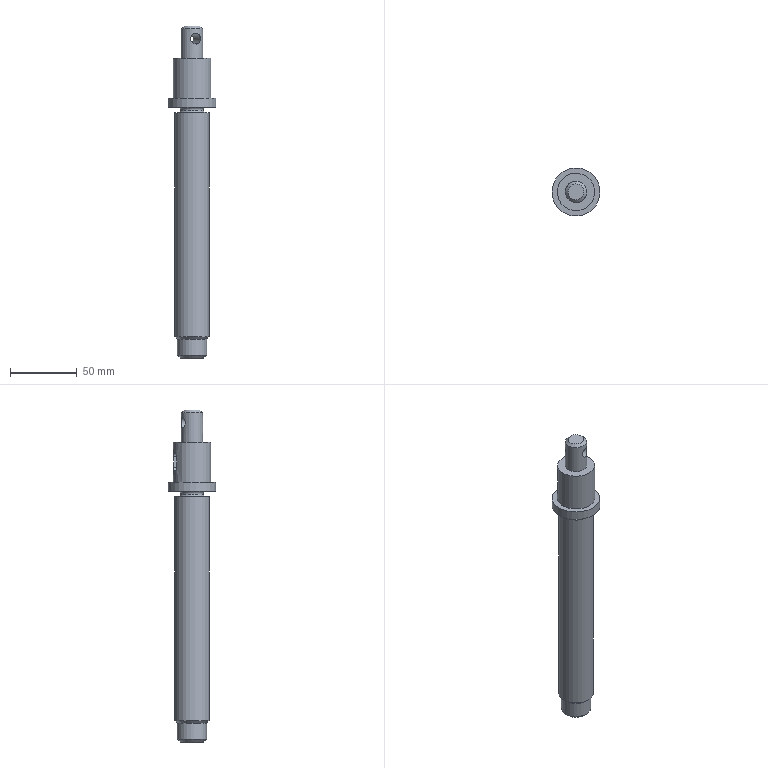Component | NX | LEADSCREW | 1 solid | 22 faces | volume 125555 mm3 | plane 9 | cylinder 8 | cone 3 | torus 2 | commonest cylinder face diameters 6 x2 16 x1 28 x1 36 x1 26 x1 22 x1 8 x1